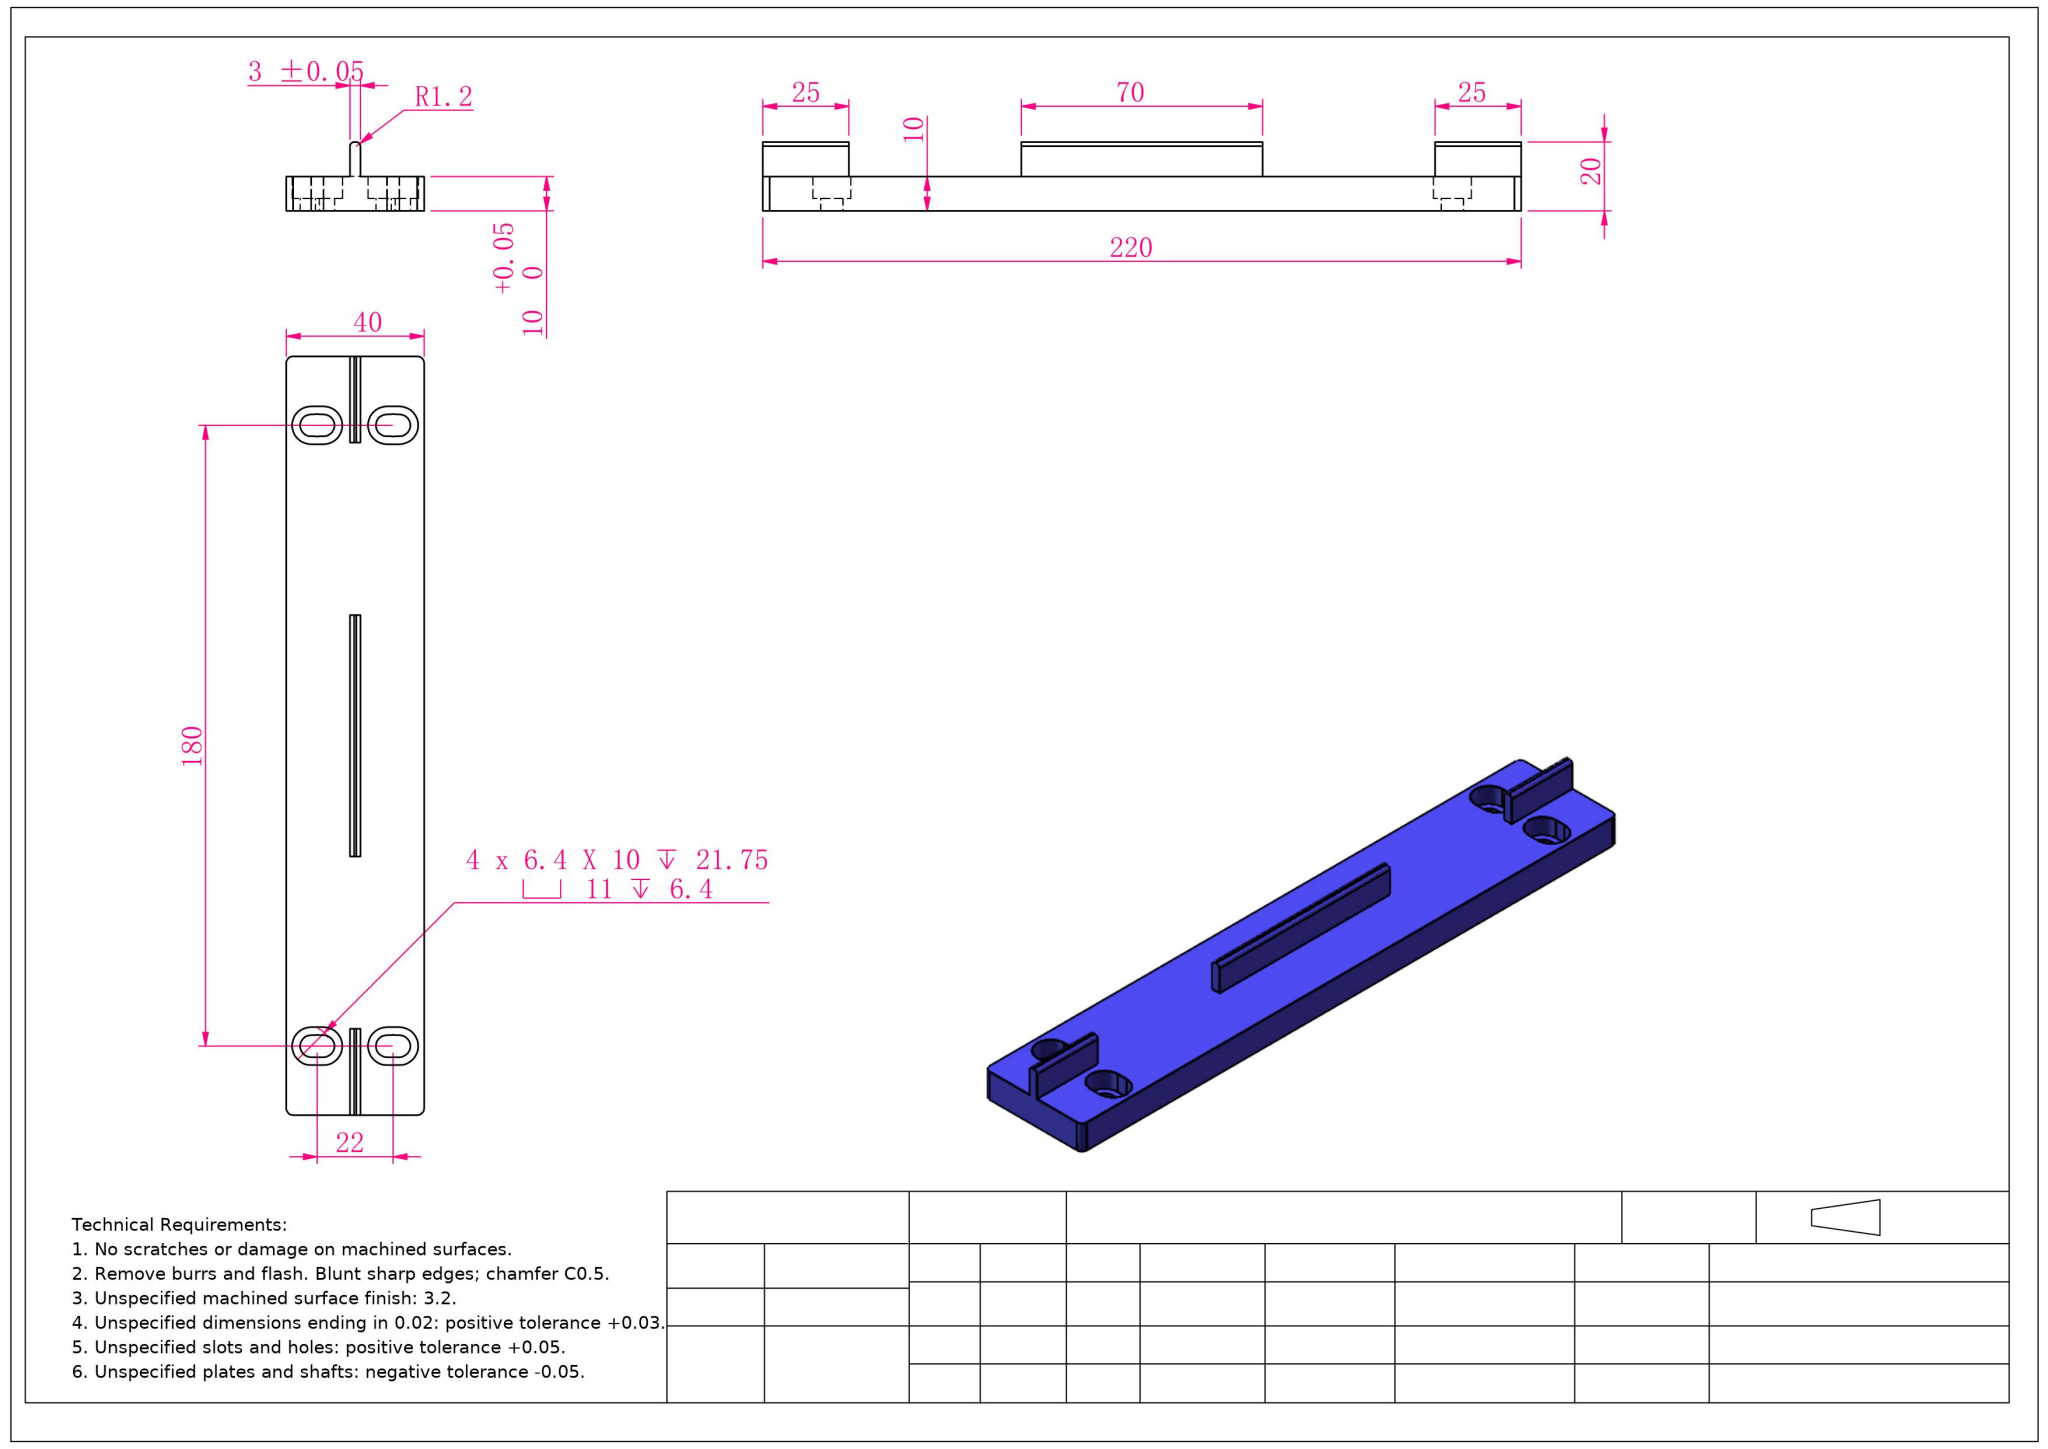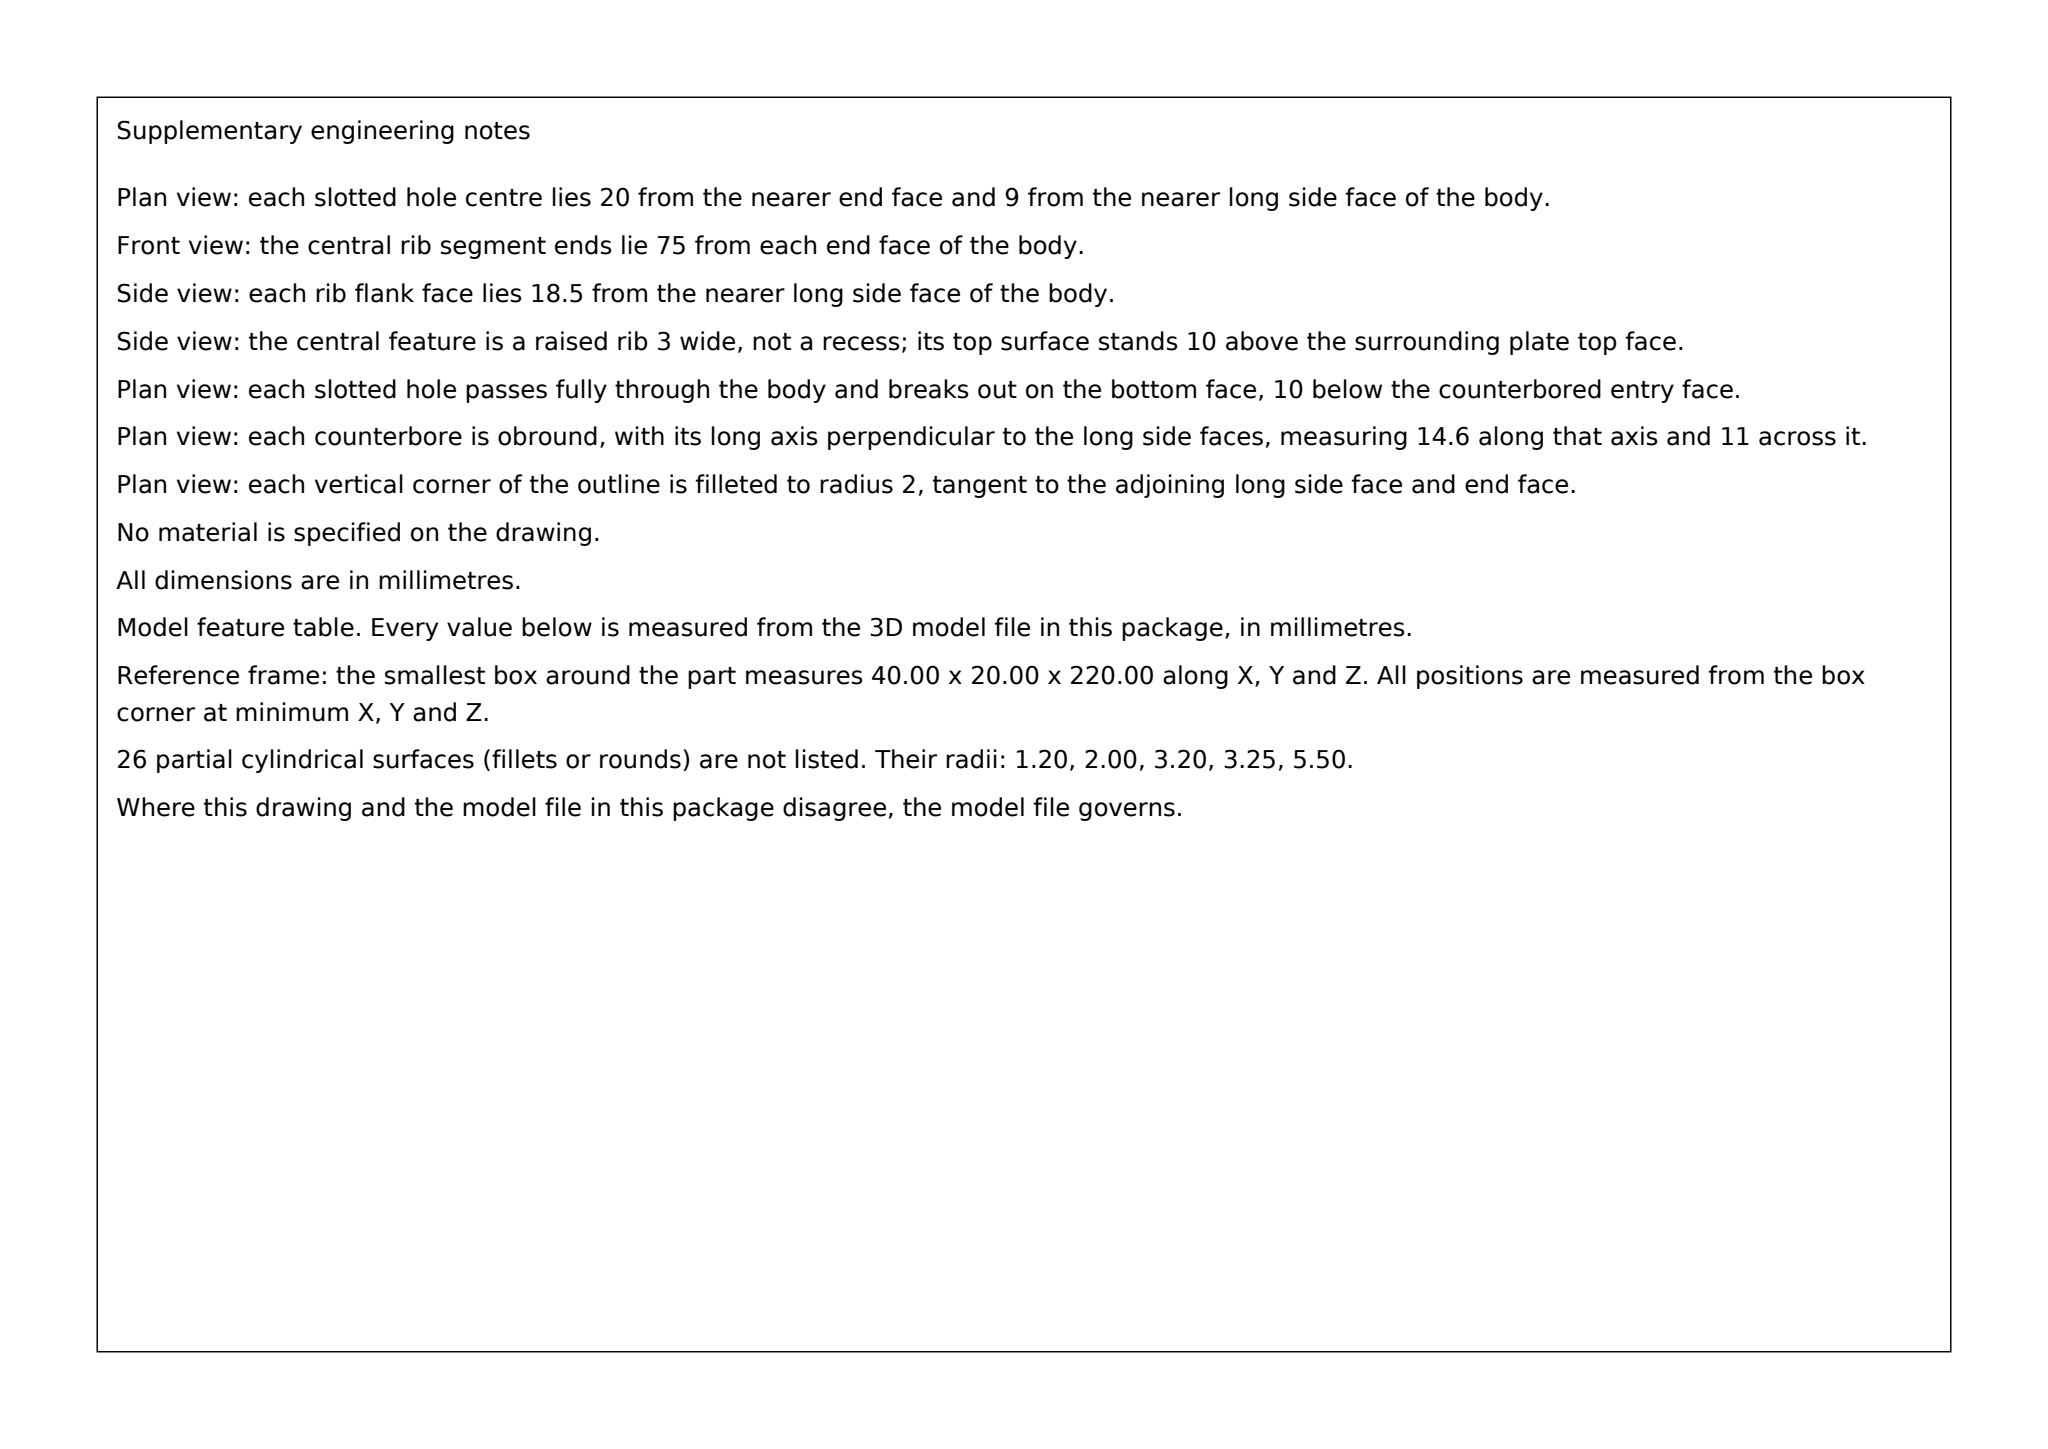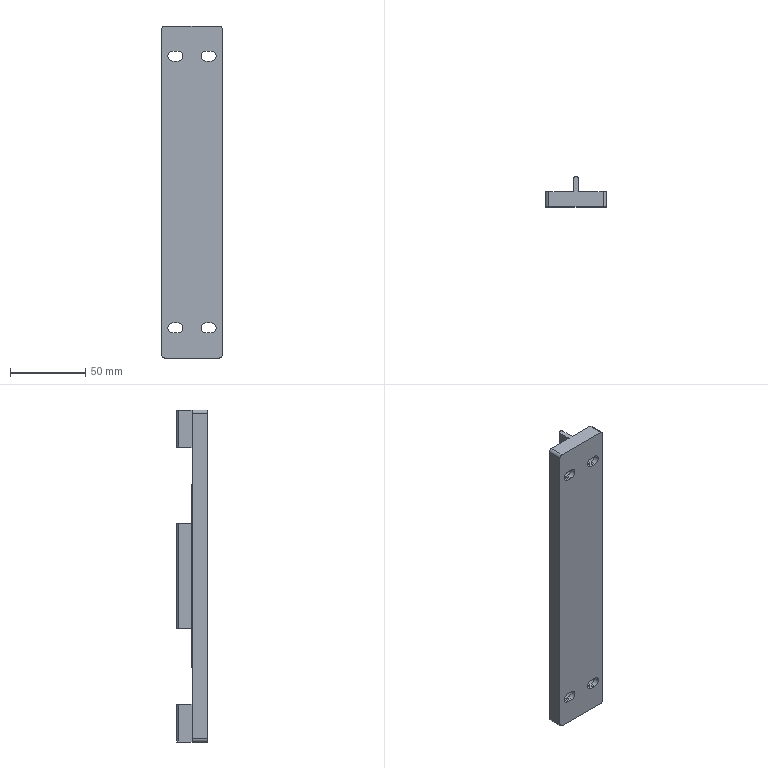Part | SolidWorks | mm | 1 solid | 81 faces | box 40 x 20 x 220 mm | volume 87249 mm3 | plane 47 | cylinder 34 | commonest cylinder face diameters 6.4 x8 11 x8 6.5 x8 2.4 x6 4 x4